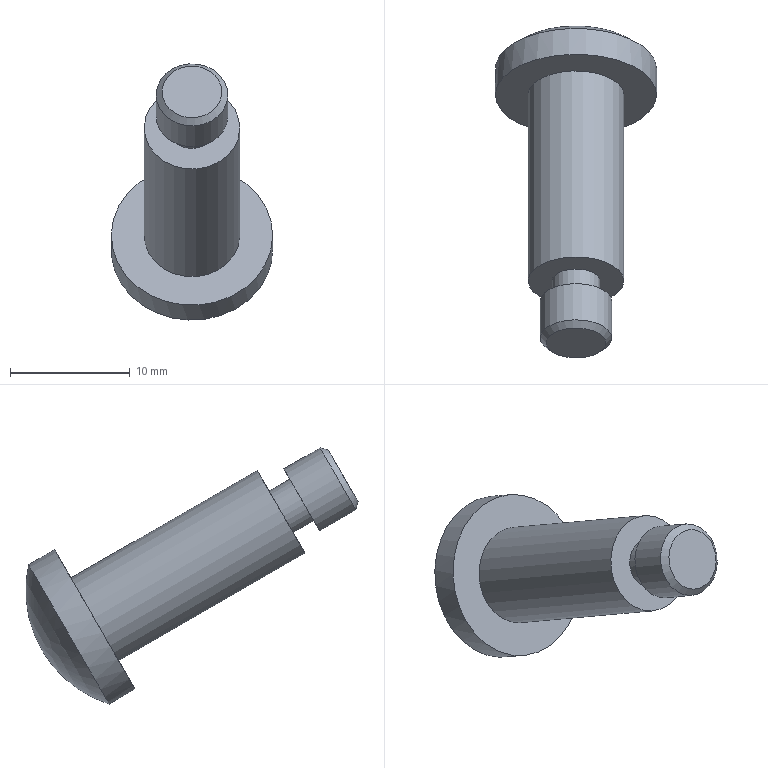Component | NX | CONNECTING_SHAFT_3 | 1 solid | 10 faces | box 13.5 x 27.81 x 21.44 mm | volume 1596 mm3 | plane 4 | cylinder 4 | cone 1 | sphere 1 | commonest cylinder face diameters 6 x1 4 x1 8 x1 13.5 x1
STEP:
#1=CARTESIAN_POINT('',(0.,0.,0.));
#2=DIRECTION('',(0.,0.,1.));
#3=DIRECTION('',(1.,0.,0.));
#4=AXIS2_PLACEMENT_3D('',#1,#2,#3);
#5=CARTESIAN_POINT('',(-8.467,14.853,-80.275));
#6=VERTEX_POINT('',#5);
#7=CARTESIAN_POINT('',(-8.293,13.856,-82.));
#8=DIRECTION('',(0.,0.866,-0.5));
#9=DIRECTION('',(-0.08716,0.4981,0.8627));
#10=AXIS2_PLACEMENT_3D('',#7,#8,#9);
#11=CIRCLE('',#10,2.);
#12=CARTESIAN_POINT('',(-8.293,13.856,-82.));
#13=DIRECTION('',(0.,0.866,-0.5));
#14=DIRECTION('',(-0.08716,0.4981,0.8627));
#15=AXIS2_PLACEMENT_3D('',#12,#13,#14);
#16=PLANE('',#15);
#17=CARTESIAN_POINT('',(0.,0.));
#18=DIRECTION('',(1.,0.));
#19=AXIS2_PLACEMENT_2D('',#17,#18);
#20=CIRCLE('',#19,2.);
#21=(GEOMETRIC_REPRESENTATION_CONTEXT(2)PARAMETRIC_REPRESENTATION_CONTEXT()REPRESENTATION_CONTEXT('',''));
#22=DEFINITIONAL_REPRESENTATION('',(#20),#21);
#23=PCURVE('',#16,#22);
#24=CARTESIAN_POINT('',(-8.293,13.856,-82.));
#25=DIRECTION('',(0.,0.866,-0.5));
#26=DIRECTION('',(-0.08716,0.4981,0.8627));
#27=AXIS2_PLACEMENT_3D('',#24,#25,#26);
#28=CYLINDRICAL_SURFACE('',#27,2.);
#29=CARTESIAN_POINT('',(0.,0.));
#30=DIRECTION('',(1.,0.));
#31=VECTOR('',#30,1.);
#32=LINE('',#29,#31);
#33=(GEOMETRIC_REPRESENTATION_CONTEXT(2)PARAMETRIC_REPRESENTATION_CONTEXT()REPRESENTATION_CONTEXT('',''));
#34=DEFINITIONAL_REPRESENTATION('',(#32),#33);
#35=PCURVE('',#28,#34);
#36=SURFACE_CURVE('',#11,(#23,#35),.PCURVE_S1.);
#37=EDGE_CURVE('',#6,#6,#36,.T.);
#38=ORIENTED_EDGE('',*,*,#37,.F.);
#39=EDGE_LOOP('',(#38));
#40=FACE_BOUND('',#39,.T.);
#41=CARTESIAN_POINT('',(-8.554,15.351,-79.412));
#42=VERTEX_POINT('',#41);
#43=CARTESIAN_POINT('',(-8.293,13.856,-82.));
#44=DIRECTION('',(-0.,-0.866,0.5));
#45=DIRECTION('',(-0.08716,0.4981,0.8627));
#46=AXIS2_PLACEMENT_3D('',#43,#44,#45);
#47=CIRCLE('',#46,3.);
#48=CARTESIAN_POINT('',(3.,-0.));
#49=CARTESIAN_POINT('',(3.,-5.196));
#50=CARTESIAN_POINT('',(-1.5,-2.598));
#51=CARTESIAN_POINT('',(-6.,0.));
#52=CARTESIAN_POINT('',(-1.5,2.598));
#53=CARTESIAN_POINT('',(3.,5.196));
#54=CARTESIAN_POINT('',(3.,-0.));
#55=(BOUNDED_CURVE()B_SPLINE_CURVE(2,(#48,#49,#50,#51,#52,#53,#54),.UNSPECIFIED.,.T.,.F.)B_SPLINE_CURVE_WITH_KNOTS((1,2,2,2,2,1),(-2.094,0.,2.094,4.189,6.283,8.378),.UNSPECIFIED.)CURVE()GEOMETRIC_REPRESENTATION_ITEM()RATIONAL_B_SPLINE_CURVE((1.,0.5,1.,0.5,1.,0.5,1.))REPRESENTATION_ITEM(''));
#56=(GEOMETRIC_REPRESENTATION_CONTEXT(2)PARAMETRIC_REPRESENTATION_CONTEXT()REPRESENTATION_CONTEXT('',''));
#57=DEFINITIONAL_REPRESENTATION('',(#55),#56);
#58=PCURVE('',#16,#57);
#59=CARTESIAN_POINT('',(-8.293,10.392,-80.));
#60=DIRECTION('',(0.,0.866,-0.5));
#61=DIRECTION('',(-0.08716,0.4981,0.8627));
#62=AXIS2_PLACEMENT_3D('',#59,#60,#61);
#63=CYLINDRICAL_SURFACE('',#62,3.);
#64=CARTESIAN_POINT('',(6.283,4.));
#65=DIRECTION('',(-1.,0.));
#66=VECTOR('',#65,1.);
#67=LINE('',#64,#66);
#68=(GEOMETRIC_REPRESENTATION_CONTEXT(2)PARAMETRIC_REPRESENTATION_CONTEXT()REPRESENTATION_CONTEXT('',''));
#69=DEFINITIONAL_REPRESENTATION('',(#67),#68);
#70=PCURVE('',#63,#69);
#71=SURFACE_CURVE('',#47,(#58,#70),.PCURVE_S1.);
#72=EDGE_CURVE('',#42,#42,#71,.T.);
#73=ORIENTED_EDGE('',*,*,#72,.F.);
#74=EDGE_LOOP('',(#73));
#75=FACE_BOUND('',#74,.T.);
#76=ADVANCED_FACE('',(#40,#75),#16,.T.);
#77=CARTESIAN_POINT('',(-8.075,9.147,-82.157));
#78=VERTEX_POINT('',#77);
#79=CARTESIAN_POINT('',(-8.293,10.392,-80.));
#80=DIRECTION('',(0.,-0.866,0.5));
#81=DIRECTION('',(0.08716,-0.4981,-0.8627));
#82=AXIS2_PLACEMENT_3D('',#79,#80,#81);
#83=CIRCLE('',#82,2.5);
#84=CARTESIAN_POINT('',(-8.293,10.392,-80.));
#85=DIRECTION('',(0.,-0.866,0.5));
#86=DIRECTION('',(0.08716,-0.4981,-0.8627));
#87=AXIS2_PLACEMENT_3D('',#84,#85,#86);
#88=PLANE('',#87);
#89=CARTESIAN_POINT('',(0.,0.));
#90=DIRECTION('',(1.,0.));
#91=AXIS2_PLACEMENT_2D('',#89,#90);
#92=CIRCLE('',#91,2.5);
#93=(GEOMETRIC_REPRESENTATION_CONTEXT(2)PARAMETRIC_REPRESENTATION_CONTEXT()REPRESENTATION_CONTEXT('',''));
#94=DEFINITIONAL_REPRESENTATION('',(#92),#93);
#95=PCURVE('',#88,#94);
#96=CARTESIAN_POINT('',(-8.293,10.825,-80.25));
#97=DIRECTION('',(0.,0.866,-0.5));
#98=DIRECTION('',(-0.08716,0.4981,0.8627));
#99=AXIS2_PLACEMENT_3D('',#96,#97,#98);
#100=CONICAL_SURFACE('',#99,3.,0.7854);
#101=CARTESIAN_POINT('',(9.425,-0.5));
#102=DIRECTION('',(-1.,0.));
#103=VECTOR('',#102,1.);
#104=LINE('',#101,#103);
#105=(GEOMETRIC_REPRESENTATION_CONTEXT(2)PARAMETRIC_REPRESENTATION_CONTEXT()REPRESENTATION_CONTEXT('',''));
#106=DEFINITIONAL_REPRESENTATION('',(#104),#105);
#107=PCURVE('',#100,#106);
#108=SURFACE_CURVE('',#83,(#95,#107),.PCURVE_S1.);
#109=EDGE_CURVE('',#78,#78,#108,.T.);
#110=ORIENTED_EDGE('',*,*,#109,.T.);
#111=EDGE_LOOP('',(#110));
#112=FACE_BOUND('',#111,.T.);
#113=ADVANCED_FACE('',(#112),#88,.T.);
#114=CARTESIAN_POINT('',(-8.031,9.331,-82.838));
#115=VERTEX_POINT('',#114);
#116=CARTESIAN_POINT('',(-8.554,12.32,-77.662));
#117=VERTEX_POINT('',#116);
#118=CARTESIAN_POINT('',(-8.293,10.825,-80.25));
#119=DIRECTION('',(0.,0.866,-0.5));
#120=DIRECTION('',(0.08716,-0.4981,-0.8627));
#121=AXIS2_PLACEMENT_3D('',#118,#119,#120);
#122=CIRCLE('',#121,3.);
#123=CARTESIAN_POINT('',(3.142,0.5));
#124=DIRECTION('',(1.,0.));
#125=VECTOR('',#124,1.);
#126=LINE('',#123,#125);
#127=(GEOMETRIC_REPRESENTATION_CONTEXT(2)PARAMETRIC_REPRESENTATION_CONTEXT()REPRESENTATION_CONTEXT('',''));
#128=DEFINITIONAL_REPRESENTATION('',(#126),#127);
#129=PCURVE('',#63,#128);
#130=CARTESIAN_POINT('',(3.142,0.));
#131=DIRECTION('',(1.,-0.));
#132=VECTOR('',#131,1.);
#133=LINE('',#130,#132);
#134=(GEOMETRIC_REPRESENTATION_CONTEXT(2)PARAMETRIC_REPRESENTATION_CONTEXT()REPRESENTATION_CONTEXT('',''));
#135=DEFINITIONAL_REPRESENTATION('',(#133),#134);
#136=PCURVE('',#100,#135);
#137=SURFACE_CURVE('',#122,(#129,#136),.PCURVE_S1.);
#138=EDGE_CURVE('',#115,#117,#137,.T.);
#139=ORIENTED_EDGE('',*,*,#138,.T.);
#140=CARTESIAN_POINT('',(-8.554,12.32,-77.662));
#141=CARTESIAN_POINT('',(-8.554,15.351,-79.412));
#142=B_SPLINE_CURVE_WITH_KNOTS('',1,(#140,#141),.UNSPECIFIED.,.F.,.F.,(2,2),(0.5,4.),.PIECEWISE_BEZIER_KNOTS.);
#143=CARTESIAN_POINT('',(6.283,0.));
#144=DIRECTION('',(0.,1.));
#145=VECTOR('',#144,1.);
#146=LINE('',#143,#145);
#147=(GEOMETRIC_REPRESENTATION_CONTEXT(2)PARAMETRIC_REPRESENTATION_CONTEXT()REPRESENTATION_CONTEXT('',''));
#148=DEFINITIONAL_REPRESENTATION('',(#146),#147);
#149=PCURVE('',#63,#148);
#150=CARTESIAN_POINT('',(0.,0.));
#151=DIRECTION('',(0.,1.));
#152=VECTOR('',#151,1.);
#153=LINE('',#150,#152);
#154=(GEOMETRIC_REPRESENTATION_CONTEXT(2)PARAMETRIC_REPRESENTATION_CONTEXT()REPRESENTATION_CONTEXT('',''));
#155=DEFINITIONAL_REPRESENTATION('',(#153),#154);
#156=PCURVE('',#63,#155);
#157=SEAM_CURVE('',#142,(#149,#156),.PCURVE_S1.);
#158=EDGE_CURVE('',#117,#42,#157,.T.);
#159=ORIENTED_EDGE('',*,*,#158,.T.);
#160=ORIENTED_EDGE('',*,*,#72,.T.);
#161=ORIENTED_EDGE('',*,*,#158,.F.);
#162=CARTESIAN_POINT('',(-8.293,10.825,-80.25));
#163=DIRECTION('',(0.,0.866,-0.5));
#164=DIRECTION('',(0.08716,-0.4981,-0.8627));
#165=AXIS2_PLACEMENT_3D('',#162,#163,#164);
#166=CIRCLE('',#165,3.);
#167=CARTESIAN_POINT('',(-3.142,0.5));
#168=DIRECTION('',(1.,0.));
#169=VECTOR('',#168,1.);
#170=LINE('',#167,#169);
#171=(GEOMETRIC_REPRESENTATION_CONTEXT(2)PARAMETRIC_REPRESENTATION_CONTEXT()REPRESENTATION_CONTEXT('',''));
#172=DEFINITIONAL_REPRESENTATION('',(#170),#171);
#173=PCURVE('',#63,#172);
#174=CARTESIAN_POINT('',(3.142,-0.));
#175=DIRECTION('',(1.,0.));
#176=VECTOR('',#175,1.);
#177=LINE('',#174,#176);
#178=(GEOMETRIC_REPRESENTATION_CONTEXT(2)PARAMETRIC_REPRESENTATION_CONTEXT()REPRESENTATION_CONTEXT('',''));
#179=DEFINITIONAL_REPRESENTATION('',(#177),#178);
#180=PCURVE('',#100,#179);
#181=SURFACE_CURVE('',#166,(#173,#180),.PCURVE_S1.);
#182=EDGE_CURVE('',#117,#115,#181,.T.);
#183=ORIENTED_EDGE('',*,*,#182,.T.);
#184=EDGE_LOOP('',(#139,#159,#160,#161,#183));
#185=FACE_BOUND('',#184,.T.);
#186=ADVANCED_FACE('',(#185),#63,.T.);
#187=ORIENTED_EDGE('',*,*,#109,.F.);
#188=CARTESIAN_POINT('',(-8.075,9.147,-82.157));
#189=CARTESIAN_POINT('',(-8.031,9.331,-82.838));
#190=B_SPLINE_CURVE_WITH_KNOTS('',1,(#188,#189),.UNSPECIFIED.,.F.,.F.,(2,2),(-0.7071,0.),.PIECEWISE_BEZIER_KNOTS.);
#191=CARTESIAN_POINT('',(9.425,0.));
#192=DIRECTION('',(0.,1.));
#193=VECTOR('',#192,1.);
#194=LINE('',#191,#193);
#195=(GEOMETRIC_REPRESENTATION_CONTEXT(2)PARAMETRIC_REPRESENTATION_CONTEXT()REPRESENTATION_CONTEXT('',''));
#196=DEFINITIONAL_REPRESENTATION('',(#194),#195);
#197=PCURVE('',#100,#196);
#198=CARTESIAN_POINT('',(3.142,0.));
#199=DIRECTION('',(0.,1.));
#200=VECTOR('',#199,1.);
#201=LINE('',#198,#200);
#202=(GEOMETRIC_REPRESENTATION_CONTEXT(2)PARAMETRIC_REPRESENTATION_CONTEXT()REPRESENTATION_CONTEXT('',''));
#203=DEFINITIONAL_REPRESENTATION('',(#201),#202);
#204=PCURVE('',#100,#203);
#205=SEAM_CURVE('',#190,(#197,#204),.PCURVE_S1.);
#206=EDGE_CURVE('',#78,#115,#205,.T.);
#207=ORIENTED_EDGE('',*,*,#206,.T.);
#208=ORIENTED_EDGE('',*,*,#182,.F.);
#209=ORIENTED_EDGE('',*,*,#138,.F.);
#210=ORIENTED_EDGE('',*,*,#206,.F.);
#211=EDGE_LOOP('',(#187,#207,#208,#209,#210));
#212=FACE_BOUND('',#211,.T.);
#213=ADVANCED_FACE('',(#212),#100,.T.);
#214=CARTESIAN_POINT('',(-8.467,16.585,-81.275));
#215=VERTEX_POINT('',#214);
#216=CARTESIAN_POINT('',(-8.293,15.588,-83.));
#217=DIRECTION('',(0.,0.866,-0.5));
#218=DIRECTION('',(-0.08716,0.4981,0.8627));
#219=AXIS2_PLACEMENT_3D('',#216,#217,#218);
#220=CIRCLE('',#219,2.);
#221=CARTESIAN_POINT('',(0.,2.));
#222=DIRECTION('',(1.,0.));
#223=VECTOR('',#222,1.);
#224=LINE('',#221,#223);
#225=(GEOMETRIC_REPRESENTATION_CONTEXT(2)PARAMETRIC_REPRESENTATION_CONTEXT()REPRESENTATION_CONTEXT('',''));
#226=DEFINITIONAL_REPRESENTATION('',(#224),#225);
#227=PCURVE('',#28,#226);
#228=CARTESIAN_POINT('',(-8.293,15.588,-83.));
#229=DIRECTION('',(0.,-0.866,0.5));
#230=DIRECTION('',(0.08716,-0.4981,-0.8627));
#231=AXIS2_PLACEMENT_3D('',#228,#229,#230);
#232=PLANE('',#231);
#233=CARTESIAN_POINT('',(-2.,-0.));
#234=CARTESIAN_POINT('',(-2.,3.464));
#235=CARTESIAN_POINT('',(1.,1.732));
#236=CARTESIAN_POINT('',(4.,0.));
#237=CARTESIAN_POINT('',(1.,-1.732));
#238=CARTESIAN_POINT('',(-2.,-3.464));
#239=CARTESIAN_POINT('',(-2.,-0.));
#240=(BOUNDED_CURVE()B_SPLINE_CURVE(2,(#233,#234,#235,#236,#237,#238,#239),.UNSPECIFIED.,.T.,.F.)B_SPLINE_CURVE_WITH_KNOTS((1,2,2,2,2,1),(-2.094,0.,2.094,4.189,6.283,8.378),.UNSPECIFIED.)CURVE()GEOMETRIC_REPRESENTATION_ITEM()RATIONAL_B_SPLINE_CURVE((1.,0.5,1.,0.5,1.,0.5,1.))REPRESENTATION_ITEM(''));
#241=(GEOMETRIC_REPRESENTATION_CONTEXT(2)PARAMETRIC_REPRESENTATION_CONTEXT()REPRESENTATION_CONTEXT('',''));
#242=DEFINITIONAL_REPRESENTATION('',(#240),#241);
#243=PCURVE('',#232,#242);
#244=SURFACE_CURVE('',#220,(#227,#243),.PCURVE_S1.);
#245=EDGE_CURVE('',#215,#215,#244,.T.);
#246=ORIENTED_EDGE('',*,*,#245,.F.);
#247=CARTESIAN_POINT('',(-8.467,14.853,-80.275));
#248=CARTESIAN_POINT('',(-8.467,16.585,-81.275));
#249=B_SPLINE_CURVE_WITH_KNOTS('',1,(#247,#248),.UNSPECIFIED.,.F.,.F.,(2,2),(0.,2.),.PIECEWISE_BEZIER_KNOTS.);
#250=CARTESIAN_POINT('',(0.,0.));
#251=DIRECTION('',(0.,1.));
#252=VECTOR('',#251,1.);
#253=LINE('',#250,#252);
#254=(GEOMETRIC_REPRESENTATION_CONTEXT(2)PARAMETRIC_REPRESENTATION_CONTEXT()REPRESENTATION_CONTEXT('',''));
#255=DEFINITIONAL_REPRESENTATION('',(#253),#254);
#256=PCURVE('',#28,#255);
#257=CARTESIAN_POINT('',(6.283,0.));
#258=DIRECTION('',(0.,1.));
#259=VECTOR('',#258,1.);
#260=LINE('',#257,#259);
#261=(GEOMETRIC_REPRESENTATION_CONTEXT(2)PARAMETRIC_REPRESENTATION_CONTEXT()REPRESENTATION_CONTEXT('',''));
#262=DEFINITIONAL_REPRESENTATION('',(#260),#261);
#263=PCURVE('',#28,#262);
#264=SEAM_CURVE('',#249,(#256,#263),.PCURVE_S1.);
#265=EDGE_CURVE('',#6,#215,#264,.T.);
#266=ORIENTED_EDGE('',*,*,#265,.F.);
#267=ORIENTED_EDGE('',*,*,#37,.T.);
#268=ORIENTED_EDGE('',*,*,#265,.T.);
#269=EDGE_LOOP('',(#246,#266,#267,#268));
#270=FACE_BOUND('',#269,.T.);
#271=ADVANCED_FACE('',(#270),#28,.T.);
#272=ORIENTED_EDGE('',*,*,#245,.T.);
#273=EDGE_LOOP('',(#272));
#274=FACE_BOUND('',#273,.T.);
#275=CARTESIAN_POINT('',(-8.641,17.581,-79.549));
#276=VERTEX_POINT('',#275);
#277=CARTESIAN_POINT('',(-8.293,15.588,-83.));
#278=DIRECTION('',(0.,0.866,-0.5));
#279=DIRECTION('',(-0.08716,0.4981,0.8627));
#280=AXIS2_PLACEMENT_3D('',#277,#278,#279);
#281=CIRCLE('',#280,4.);
#282=CARTESIAN_POINT('',(-4.,-0.));
#283=CARTESIAN_POINT('',(-4.,6.928));
#284=CARTESIAN_POINT('',(2.,3.464));
#285=CARTESIAN_POINT('',(8.,0.));
#286=CARTESIAN_POINT('',(2.,-3.464));
#287=CARTESIAN_POINT('',(-4.,-6.928));
#288=CARTESIAN_POINT('',(-4.,-0.));
#289=(BOUNDED_CURVE()B_SPLINE_CURVE(2,(#282,#283,#284,#285,#286,#287,#288),.UNSPECIFIED.,.T.,.F.)B_SPLINE_CURVE_WITH_KNOTS((1,2,2,2,2,1),(-2.094,0.,2.094,4.189,6.283,8.378),.UNSPECIFIED.)CURVE()GEOMETRIC_REPRESENTATION_ITEM()RATIONAL_B_SPLINE_CURVE((1.,0.5,1.,0.5,1.,0.5,1.))REPRESENTATION_ITEM(''));
#290=(GEOMETRIC_REPRESENTATION_CONTEXT(2)PARAMETRIC_REPRESENTATION_CONTEXT()REPRESENTATION_CONTEXT('',''));
#291=DEFINITIONAL_REPRESENTATION('',(#289),#290);
#292=PCURVE('',#232,#291);
#293=CARTESIAN_POINT('',(-8.293,15.588,-83.));
#294=DIRECTION('',(0.,0.866,-0.5));
#295=DIRECTION('',(-0.08716,0.4981,0.8627));
#296=AXIS2_PLACEMENT_3D('',#293,#294,#295);
#297=CYLINDRICAL_SURFACE('',#296,4.);
#298=CARTESIAN_POINT('',(0.,0.));
#299=DIRECTION('',(1.,0.));
#300=VECTOR('',#299,1.);
#301=LINE('',#298,#300);
#302=(GEOMETRIC_REPRESENTATION_CONTEXT(2)PARAMETRIC_REPRESENTATION_CONTEXT()REPRESENTATION_CONTEXT('',''));
#303=DEFINITIONAL_REPRESENTATION('',(#301),#302);
#304=PCURVE('',#297,#303);
#305=SURFACE_CURVE('',#281,(#292,#304),.PCURVE_S1.);
#306=EDGE_CURVE('',#276,#276,#305,.T.);
#307=ORIENTED_EDGE('',*,*,#306,.F.);
#308=EDGE_LOOP('',(#307));
#309=FACE_BOUND('',#308,.T.);
#310=ADVANCED_FACE('',(#274,#309),#232,.T.);
#311=CARTESIAN_POINT('',(-8.641,33.169,-88.549));
#312=VERTEX_POINT('',#311);
#313=CARTESIAN_POINT('',(-8.293,31.177,-92.));
#314=DIRECTION('',(0.,0.866,-0.5));
#315=DIRECTION('',(-0.08716,0.4981,0.8627));
#316=AXIS2_PLACEMENT_3D('',#313,#314,#315);
#317=CIRCLE('',#316,4.);
#318=CARTESIAN_POINT('',(0.,18.));
#319=DIRECTION('',(1.,0.));
#320=VECTOR('',#319,1.);
#321=LINE('',#318,#320);
#322=(GEOMETRIC_REPRESENTATION_CONTEXT(2)PARAMETRIC_REPRESENTATION_CONTEXT()REPRESENTATION_CONTEXT('',''));
#323=DEFINITIONAL_REPRESENTATION('',(#321),#322);
#324=PCURVE('',#297,#323);
#325=CARTESIAN_POINT('',(-8.293,31.177,-92.));
#326=DIRECTION('',(0.,-0.866,0.5));
#327=DIRECTION('',(0.08716,-0.4981,-0.8627));
#328=AXIS2_PLACEMENT_3D('',#325,#326,#327);
#329=PLANE('',#328);
#330=CARTESIAN_POINT('',(-4.,-0.));
#331=CARTESIAN_POINT('',(-4.,6.928));
#332=CARTESIAN_POINT('',(2.,3.464));
#333=CARTESIAN_POINT('',(8.,0.));
#334=CARTESIAN_POINT('',(2.,-3.464));
#335=CARTESIAN_POINT('',(-4.,-6.928));
#336=CARTESIAN_POINT('',(-4.,-0.));
#337=(BOUNDED_CURVE()B_SPLINE_CURVE(2,(#330,#331,#332,#333,#334,#335,#336),.UNSPECIFIED.,.T.,.F.)B_SPLINE_CURVE_WITH_KNOTS((1,2,2,2,2,1),(-2.094,0.,2.094,4.189,6.283,8.378),.UNSPECIFIED.)CURVE()GEOMETRIC_REPRESENTATION_ITEM()RATIONAL_B_SPLINE_CURVE((1.,0.5,1.,0.5,1.,0.5,1.))REPRESENTATION_ITEM(''));
#338=(GEOMETRIC_REPRESENTATION_CONTEXT(2)PARAMETRIC_REPRESENTATION_CONTEXT()REPRESENTATION_CONTEXT('',''));
#339=DEFINITIONAL_REPRESENTATION('',(#337),#338);
#340=PCURVE('',#329,#339);
#341=SURFACE_CURVE('',#317,(#324,#340),.PCURVE_S1.);
#342=EDGE_CURVE('',#312,#312,#341,.T.);
#343=ORIENTED_EDGE('',*,*,#342,.F.);
#344=CARTESIAN_POINT('',(-8.641,17.581,-79.549));
#345=CARTESIAN_POINT('',(-8.641,33.169,-88.549));
#346=B_SPLINE_CURVE_WITH_KNOTS('',1,(#344,#345),.UNSPECIFIED.,.F.,.F.,(2,2),(0.,18.),.PIECEWISE_BEZIER_KNOTS.);
#347=CARTESIAN_POINT('',(0.,0.));
#348=DIRECTION('',(0.,1.));
#349=VECTOR('',#348,1.);
#350=LINE('',#347,#349);
#351=(GEOMETRIC_REPRESENTATION_CONTEXT(2)PARAMETRIC_REPRESENTATION_CONTEXT()REPRESENTATION_CONTEXT('',''));
#352=DEFINITIONAL_REPRESENTATION('',(#350),#351);
#353=PCURVE('',#297,#352);
#354=CARTESIAN_POINT('',(6.283,0.));
#355=DIRECTION('',(0.,1.));
#356=VECTOR('',#355,1.);
#357=LINE('',#354,#356);
#358=(GEOMETRIC_REPRESENTATION_CONTEXT(2)PARAMETRIC_REPRESENTATION_CONTEXT()REPRESENTATION_CONTEXT('',''));
#359=DEFINITIONAL_REPRESENTATION('',(#357),#358);
#360=PCURVE('',#297,#359);
#361=SEAM_CURVE('',#346,(#353,#360),.PCURVE_S1.);
#362=EDGE_CURVE('',#276,#312,#361,.T.);
#363=ORIENTED_EDGE('',*,*,#362,.F.);
#364=ORIENTED_EDGE('',*,*,#306,.T.);
#365=ORIENTED_EDGE('',*,*,#362,.T.);
#366=EDGE_LOOP('',(#343,#363,#364,#365));
#367=FACE_BOUND('',#366,.T.);
#368=ADVANCED_FACE('',(#367),#297,.T.);
#369=ORIENTED_EDGE('',*,*,#342,.T.);
#370=EDGE_LOOP('',(#369));
#371=FACE_BOUND('',#370,.T.);
#372=CARTESIAN_POINT('',(-8.881,34.539,-86.177));
#373=VERTEX_POINT('',#372);
#374=CARTESIAN_POINT('',(-8.293,31.177,-92.));
#375=DIRECTION('',(0.,0.866,-0.5));
#376=DIRECTION('',(-0.08716,0.4981,0.8627));
#377=AXIS2_PLACEMENT_3D('',#374,#375,#376);
#378=CIRCLE('',#377,6.75);
#379=CARTESIAN_POINT('',(-6.75,0.));
#380=CARTESIAN_POINT('',(-6.75,11.691));
#381=CARTESIAN_POINT('',(3.375,5.846));
#382=CARTESIAN_POINT('',(13.5,0.));
#383=CARTESIAN_POINT('',(3.375,-5.846));
#384=CARTESIAN_POINT('',(-6.75,-11.691));
#385=CARTESIAN_POINT('',(-6.75,0.));
#386=(BOUNDED_CURVE()B_SPLINE_CURVE(2,(#379,#380,#381,#382,#383,#384,#385),.UNSPECIFIED.,.T.,.F.)B_SPLINE_CURVE_WITH_KNOTS((1,2,2,2,2,1),(-2.094,0.,2.094,4.189,6.283,8.378),.UNSPECIFIED.)CURVE()GEOMETRIC_REPRESENTATION_ITEM()RATIONAL_B_SPLINE_CURVE((1.,0.5,1.,0.5,1.,0.5,1.))REPRESENTATION_ITEM(''));
#387=(GEOMETRIC_REPRESENTATION_CONTEXT(2)PARAMETRIC_REPRESENTATION_CONTEXT()REPRESENTATION_CONTEXT('',''));
#388=DEFINITIONAL_REPRESENTATION('',(#386),#387);
#389=PCURVE('',#329,#388);
#390=CARTESIAN_POINT('',(-8.293,31.177,-92.));
#391=DIRECTION('',(0.,0.866,-0.5));
#392=DIRECTION('',(-0.08716,0.4981,0.8627));
#393=AXIS2_PLACEMENT_3D('',#390,#391,#392);
#394=CYLINDRICAL_SURFACE('',#393,6.75);
#395=CARTESIAN_POINT('',(0.,0.));
#396=DIRECTION('',(1.,0.));
#397=VECTOR('',#396,1.);
#398=LINE('',#395,#397);
#399=(GEOMETRIC_REPRESENTATION_CONTEXT(2)PARAMETRIC_REPRESENTATION_CONTEXT()REPRESENTATION_CONTEXT('',''));
#400=DEFINITIONAL_REPRESENTATION('',(#398),#399);
#401=PCURVE('',#394,#400);
#402=SURFACE_CURVE('',#378,(#389,#401),.PCURVE_S1.);
#403=EDGE_CURVE('',#373,#373,#402,.T.);
#404=ORIENTED_EDGE('',*,*,#403,.F.);
#405=EDGE_LOOP('',(#404));
#406=FACE_BOUND('',#405,.T.);
#407=ADVANCED_FACE('',(#371,#406),#329,.T.);
#408=CARTESIAN_POINT('',(-8.881,36.704,-87.427));
#409=VERTEX_POINT('',#408);
#410=CARTESIAN_POINT('',(-15.017,33.048,-93.759));
#411=VERTEX_POINT('',#410);
#412=CARTESIAN_POINT('',(-8.293,33.342,-93.25));
#413=DIRECTION('',(0.,0.866,-0.5));
#414=DIRECTION('',(-0.08716,0.4981,0.8627));
#415=AXIS2_PLACEMENT_3D('',#412,#413,#414);
#416=CIRCLE('',#415,6.75);
#417=CARTESIAN_POINT('',(0.,2.5));
#418=DIRECTION('',(1.,0.));
#419=VECTOR('',#418,1.);
#420=LINE('',#417,#419);
#421=(GEOMETRIC_REPRESENTATION_CONTEXT(2)PARAMETRIC_REPRESENTATION_CONTEXT()REPRESENTATION_CONTEXT('',''));
#422=DEFINITIONAL_REPRESENTATION('',(#420),#421);
#423=PCURVE('',#394,#422);
#424=CARTESIAN_POINT('',(-8.293,26.952,-89.561));
#425=DIRECTION('',(0.,0.866,-0.5));
#426=DIRECTION('',(-0.9962,-0.04358,-0.07548));
#427=AXIS2_PLACEMENT_3D('',#424,#425,#426);
#428=SPHERICAL_SURFACE('',#427,10.);
#429=CARTESIAN_POINT('',(1.571,0.8298));
#430=CARTESIAN_POINT('',(1.666,0.8298));
#431=CARTESIAN_POINT('',(1.856,0.8298));
#432=CARTESIAN_POINT('',(2.142,0.8298));
#433=CARTESIAN_POINT('',(2.428,0.8298));
#434=CARTESIAN_POINT('',(2.713,0.8298));
#435=CARTESIAN_POINT('',(2.999,0.8298));
#436=CARTESIAN_POINT('',(3.284,0.8298));
#437=CARTESIAN_POINT('',(3.57,0.8298));
#438=CARTESIAN_POINT('',(3.856,0.8298));
#439=CARTESIAN_POINT('',(4.141,0.8298));
#440=CARTESIAN_POINT('',(4.427,0.8298));
#441=CARTESIAN_POINT('',(4.712,0.8298));
#442=CARTESIAN_POINT('',(4.998,0.8298));
#443=CARTESIAN_POINT('',(5.284,0.8298));
#444=CARTESIAN_POINT('',(5.569,0.8298));
#445=CARTESIAN_POINT('',(5.855,0.8298));
#446=CARTESIAN_POINT('',(6.14,0.8298));
#447=CARTESIAN_POINT('',(6.426,0.8298));
#448=CARTESIAN_POINT('',(6.712,0.8298));
#449=CARTESIAN_POINT('',(6.997,0.8298));
#450=CARTESIAN_POINT('',(7.283,0.8298));
#451=CARTESIAN_POINT('',(7.568,0.8298));
#452=CARTESIAN_POINT('',(7.759,0.8298));
#453=CARTESIAN_POINT('',(7.854,0.8298));
#454=B_SPLINE_CURVE_WITH_KNOTS('',3,(#429,#430,#431,#432,#433,#434,#435,#436,#437,#438,#439,#440,#441,#442,#443,#444,#445,#446,#447,#448,#449,#450,#451,#452,#453),.UNSPECIFIED.,.F.,.F.,(4,1,1,1,1,1,1,1,1,1,1,1,1,1,1,1,1,1,1,1,1,1,4),(0.,0.2856,0.5712,0.8568,1.142,1.428,1.714,1.999,2.285,2.57,2.856,3.142,3.427,3.713,3.998,4.284,4.57,4.855,5.141,5.426,5.712,5.998,6.283),.QUASI_UNIFORM_KNOTS.);
#455=(GEOMETRIC_REPRESENTATION_CONTEXT(2)PARAMETRIC_REPRESENTATION_CONTEXT()REPRESENTATION_CONTEXT('',''));
#456=DEFINITIONAL_REPRESENTATION('',(#454),#455);
#457=PCURVE('',#428,#456);
#458=SURFACE_CURVE('',#416,(#423,#457),.PCURVE_S1.);
#459=EDGE_CURVE('',#409,#411,#458,.T.);
#460=ORIENTED_EDGE('',*,*,#459,.F.);
#461=CARTESIAN_POINT('',(-8.881,34.539,-86.177));
#462=CARTESIAN_POINT('',(-8.881,36.704,-87.427));
#463=B_SPLINE_CURVE_WITH_KNOTS('',1,(#461,#462),.UNSPECIFIED.,.F.,.F.,(2,2),(0.,2.5),.PIECEWISE_BEZIER_KNOTS.);
#464=CARTESIAN_POINT('',(0.,0.));
#465=DIRECTION('',(0.,1.));
#466=VECTOR('',#465,1.);
#467=LINE('',#464,#466);
#468=(GEOMETRIC_REPRESENTATION_CONTEXT(2)PARAMETRIC_REPRESENTATION_CONTEXT()REPRESENTATION_CONTEXT('',''));
#469=DEFINITIONAL_REPRESENTATION('',(#467),#468);
#470=PCURVE('',#394,#469);
#471=CARTESIAN_POINT('',(6.283,0.));
#472=DIRECTION('',(0.,1.));
#473=VECTOR('',#472,1.);
#474=LINE('',#471,#473);
#475=(GEOMETRIC_REPRESENTATION_CONTEXT(2)PARAMETRIC_REPRESENTATION_CONTEXT()REPRESENTATION_CONTEXT('',''));
#476=DEFINITIONAL_REPRESENTATION('',(#474),#475);
#477=PCURVE('',#394,#476);
#478=SEAM_CURVE('',#463,(#470,#477),.PCURVE_S1.);
#479=EDGE_CURVE('',#373,#409,#478,.T.);
#480=ORIENTED_EDGE('',*,*,#479,.F.);
#481=ORIENTED_EDGE('',*,*,#403,.T.);
#482=ORIENTED_EDGE('',*,*,#479,.T.);
#483=CARTESIAN_POINT('',(-8.293,33.342,-93.25));
#484=DIRECTION('',(0.,0.866,-0.5));
#485=DIRECTION('',(-0.08716,0.4981,0.8627));
#486=AXIS2_PLACEMENT_3D('',#483,#484,#485);
#487=CIRCLE('',#486,6.75);
#488=CARTESIAN_POINT('',(0.,2.5));
#489=DIRECTION('',(1.,0.));
#490=VECTOR('',#489,1.);
#491=LINE('',#488,#490);
#492=(GEOMETRIC_REPRESENTATION_CONTEXT(2)PARAMETRIC_REPRESENTATION_CONTEXT()REPRESENTATION_CONTEXT('',''));
#493=DEFINITIONAL_REPRESENTATION('',(#491),#492);
#494=PCURVE('',#394,#493);
#495=CARTESIAN_POINT('',(-4.712,0.8298));
#496=CARTESIAN_POINT('',(-4.617,0.8298));
#497=CARTESIAN_POINT('',(-4.427,0.8298));
#498=CARTESIAN_POINT('',(-4.141,0.8298));
#499=CARTESIAN_POINT('',(-3.856,0.8298));
#500=CARTESIAN_POINT('',(-3.57,0.8298));
#501=CARTESIAN_POINT('',(-3.284,0.8298));
#502=CARTESIAN_POINT('',(-2.999,0.8298));
#503=CARTESIAN_POINT('',(-2.713,0.8298));
#504=CARTESIAN_POINT('',(-2.428,0.8298));
#505=CARTESIAN_POINT('',(-2.142,0.8298));
#506=CARTESIAN_POINT('',(-1.856,0.8298));
#507=CARTESIAN_POINT('',(-1.571,0.8298));
#508=CARTESIAN_POINT('',(-1.285,0.8298));
#509=CARTESIAN_POINT('',(-0.9996,0.8298));
#510=CARTESIAN_POINT('',(-0.714,0.8298));
#511=CARTESIAN_POINT('',(-0.4284,0.8298));
#512=CARTESIAN_POINT('',(-0.1428,0.8298));
#513=CARTESIAN_POINT('',(0.1428,0.8298));
#514=CARTESIAN_POINT('',(0.4284,0.8298));
#515=CARTESIAN_POINT('',(0.714,0.8298));
#516=CARTESIAN_POINT('',(0.9996,0.8298));
#517=CARTESIAN_POINT('',(1.285,0.8298));
#518=CARTESIAN_POINT('',(1.476,0.8298));
#519=CARTESIAN_POINT('',(1.571,0.8298));
#520=B_SPLINE_CURVE_WITH_KNOTS('',3,(#495,#496,#497,#498,#499,#500,#501,#502,#503,#504,#505,#506,#507,#508,#509,#510,#511,#512,#513,#514,#515,#516,#517,#518,#519),.UNSPECIFIED.,.F.,.F.,(4,1,1,1,1,1,1,1,1,1,1,1,1,1,1,1,1,1,1,1,1,1,4),(0.,0.2856,0.5712,0.8568,1.142,1.428,1.714,1.999,2.285,2.57,2.856,3.142,3.427,3.713,3.998,4.284,4.57,4.855,5.141,5.426,5.712,5.998,6.283),.QUASI_UNIFORM_KNOTS.);
#521=(GEOMETRIC_REPRESENTATION_CONTEXT(2)PARAMETRIC_REPRESENTATION_CONTEXT()REPRESENTATION_CONTEXT('',''));
#522=DEFINITIONAL_REPRESENTATION('',(#520),#521);
#523=PCURVE('',#428,#522);
#524=SURFACE_CURVE('',#487,(#494,#523),.PCURVE_S1.);
#525=EDGE_CURVE('',#411,#409,#524,.T.);
#526=ORIENTED_EDGE('',*,*,#525,.F.);
#527=EDGE_LOOP('',(#460,#480,#481,#482,#526));
#528=FACE_BOUND('',#527,.T.);
#529=ADVANCED_FACE('',(#528),#394,.T.);
#530=ORIENTED_EDGE('',*,*,#459,.T.);
#531=CARTESIAN_POINT('',(-8.293,35.613,-94.561));
#532=VERTEX_POINT('',#531);
#533=CARTESIAN_POINT('',(-15.017,33.048,-93.759));
#534=CARTESIAN_POINT('',(-13.928,33.962,-94.177));
#535=CARTESIAN_POINT('',(-12.654,34.708,-94.479));
#536=CARTESIAN_POINT('',(-11.245,35.246,-94.647));
#537=CARTESIAN_POINT('',(-9.769,35.548,-94.673));
#538=CARTESIAN_POINT('',(-8.293,35.613,-94.561));
#539=B_SPLINE_CURVE_WITH_KNOTS('',5,(#533,#534,#535,#536,#537,#538),.UNSPECIFIED.,.F.,.F.,(6,6),(0.8298,1.571),.PIECEWISE_BEZIER_KNOTS.);
#540=CARTESIAN_POINT('',(6.283,0.));
#541=DIRECTION('',(0.,1.));
#542=VECTOR('',#541,1.);
#543=LINE('',#540,#542);
#544=(GEOMETRIC_REPRESENTATION_CONTEXT(2)PARAMETRIC_REPRESENTATION_CONTEXT()REPRESENTATION_CONTEXT('',''));
#545=DEFINITIONAL_REPRESENTATION('',(#543),#544);
#546=PCURVE('',#428,#545);
#547=CARTESIAN_POINT('',(0.,0.));
#548=DIRECTION('',(0.,1.));
#549=VECTOR('',#548,1.);
#550=LINE('',#547,#549);
#551=(GEOMETRIC_REPRESENTATION_CONTEXT(2)PARAMETRIC_REPRESENTATION_CONTEXT()REPRESENTATION_CONTEXT('',''));
#552=DEFINITIONAL_REPRESENTATION('',(#550),#551);
#553=PCURVE('',#428,#552);
#554=SEAM_CURVE('',#539,(#546,#553),.PCURVE_S1.);
#555=EDGE_CURVE('',#411,#532,#554,.T.);
#556=ORIENTED_EDGE('',*,*,#555,.T.);
#557=ORIENTED_EDGE('',*,*,#555,.F.);
#558=ORIENTED_EDGE('',*,*,#525,.T.);
#559=EDGE_LOOP('',(#530,#556,#557,#558));
#560=FACE_BOUND('',#559,.T.);
#561=ADVANCED_FACE('',(#560),#428,.T.);
#562=CLOSED_SHELL('',(#76,#113,#186,#213,#271,#310,#368,#407,#529,#561));
#563=MANIFOLD_SOLID_BREP('',#562);
#564=(LENGTH_UNIT()NAMED_UNIT(*)SI_UNIT(.MILLI.,.METRE.));
#565=UNCERTAINTY_MEASURE_WITH_UNIT(LENGTH_MEASURE(0.00001),#564,'','');
#566=(NAMED_UNIT(*)PLANE_ANGLE_UNIT()SI_UNIT($,.RADIAN.));
#567=(NAMED_UNIT(*)SI_UNIT($,.STERADIAN.)SOLID_ANGLE_UNIT());
#568=(GEOMETRIC_REPRESENTATION_CONTEXT(3)GLOBAL_UNCERTAINTY_ASSIGNED_CONTEXT((#565))GLOBAL_UNIT_ASSIGNED_CONTEXT((#564,#566,#567))REPRESENTATION_CONTEXT('',''));
#569=ADVANCED_BREP_SHAPE_REPRESENTATION('',(#4,#563),#568);